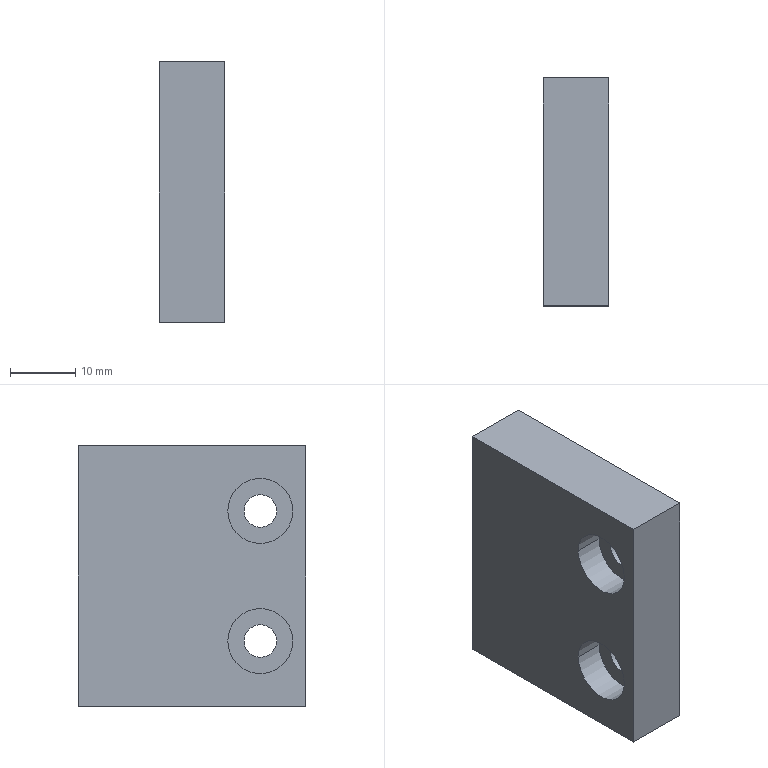Component | SolidWorks | SYM0545-81-107-2 | 1 solid | 16 faces | box 10 x 35 x 40 mm | volume 13077 mm3 | cylinder 8 | plane 8 | commonest cylinder face diameters 10 x4 5 x4 | material PP Copolymer
build123d program:
from build123d import *

# Parameters (mm, degrees)
SKETCH2_W       = 40
SKETCH2_H       = 35
EXTRUDE1_DEPTH  = 10
SKETCH3_R       = 2.5
EXTRUDE3_DEPTH  = 42.533
SKETCH4_R       = 5
EXTRUDE4_DEPTH  = 4.5
LPATTERN1_COUNT = 2
LPATTERN1_PITCH = 20


with BuildPart() as part:
    # Sketch2 → Extrude1 (new body)
    with BuildSketch(Plane(origin=(0, 0, 0), x_dir=(1, 0, 0), z_dir=(0, 1, 0))):
        with Locations((0, -17.5)):
            Rectangle(SKETCH2_W, SKETCH2_H)
    extrude(amount=EXTRUDE1_DEPTH)

    # Sketch3 → Extrude3 (cut, through all)
    with BuildSketch(Plane(origin=(0, 0, 0), x_dir=(1, 0, 0), z_dir=(0, 1, 0))):
        with Locations(Location((-10, -28, 0), (0, 0, 270))):
            Circle(SKETCH3_R)
    extrude3 = extrude(amount=EXTRUDE3_DEPTH, mode=Mode.SUBTRACT)

    # Sketch4 → Extrude4 (cut)
    with BuildSketch(Plane(origin=(0, 10, 0), x_dir=(1, 0, 0), z_dir=(0, 1, 0))):
        with Locations(Location((-10, -28, 0), (0, 0, 270))):
            Circle(SKETCH4_R)
    extrude4 = extrude(amount=-EXTRUDE4_DEPTH, mode=Mode.SUBTRACT)

    # LPattern1: Extrude3, Extrude4 ×2
    with Locations(*[(i * LPATTERN1_PITCH, 0, 0) for i in range(1, LPATTERN1_COUNT)]):
        add(extrude3, mode=Mode.SUBTRACT)
        add(extrude4, mode=Mode.SUBTRACT)


solid = part.part

# Placed as in the assembly
solid = solid.moved(Location((322.251, 468.143, 1010.518), (90, 0, 90)))
STEP:
#1=CARTESIAN_POINT('',(12.471,17.525,40.178));
#2=VERTEX_POINT('',#1);
#3=CARTESIAN_POINT('',(12.471,17.132,40.178));
#4=VERTEX_POINT('',#3);
#5=CARTESIAN_POINT('',(12.471,17.328,40.178));
#6=DIRECTION('',(-1.,0.,0.));
#7=DIRECTION('',(0.,-1.,0.));
#8=AXIS2_PLACEMENT_3D('',#5,#6,#7);
#9=CIRCLE('',#8,0.1969);
#10=EDGE_CURVE('',#2,#4,#9,.T.);
#11=ORIENTED_EDGE('',*,*,#10,.F.);
#12=CARTESIAN_POINT('',(12.293,17.525,40.178));
#13=VERTEX_POINT('',#12);
#14=CARTESIAN_POINT('',(12.471,17.525,40.178));
#15=DIRECTION('',(-1.,0.,0.));
#16=VECTOR('',#15,39.37);
#17=LINE('',#14,#16);
#18=EDGE_CURVE('',#2,#13,#17,.T.);
#19=ORIENTED_EDGE('',*,*,#18,.T.);
#20=CARTESIAN_POINT('',(12.293,17.132,40.178));
#21=VERTEX_POINT('',#20);
#22=CARTESIAN_POINT('',(12.293,17.328,40.178));
#23=DIRECTION('',(-1.,0.,0.));
#24=DIRECTION('',(0.,-1.,0.));
#25=AXIS2_PLACEMENT_3D('',#22,#23,#24);
#26=CIRCLE('',#25,0.1969);
#27=EDGE_CURVE('',#13,#21,#26,.T.);
#28=ORIENTED_EDGE('',*,*,#27,.T.);
#29=CARTESIAN_POINT('',(12.471,17.132,40.178));
#30=DIRECTION('',(-1.,0.,0.));
#31=VECTOR('',#30,39.37);
#32=LINE('',#29,#31);
#33=EDGE_CURVE('',#4,#21,#32,.T.);
#34=ORIENTED_EDGE('',*,*,#33,.F.);
#35=EDGE_LOOP('',(#11,#19,#28,#34));
#36=FACE_OUTER_BOUND('',#35,.T.);
#37=CARTESIAN_POINT('',(12.471,17.328,40.178));
#38=DIRECTION('',(-1.,0.,0.));
#39=DIRECTION('',(0.,-1.,0.));
#40=AXIS2_PLACEMENT_3D('',#37,#38,#39);
#41=CYLINDRICAL_SURFACE('',#40,0.1969);
#42=ADVANCED_FACE('',(#36),#41,.F.);
#43=CARTESIAN_POINT('',(12.471,17.525,39.39));
#44=VERTEX_POINT('',#43);
#45=CARTESIAN_POINT('',(12.471,17.132,39.39));
#46=VERTEX_POINT('',#45);
#47=CARTESIAN_POINT('',(12.471,17.328,39.39));
#48=DIRECTION('',(-1.,0.,0.));
#49=DIRECTION('',(0.,-1.,0.));
#50=AXIS2_PLACEMENT_3D('',#47,#48,#49);
#51=CIRCLE('',#50,0.1969);
#52=EDGE_CURVE('',#44,#46,#51,.T.);
#53=ORIENTED_EDGE('',*,*,#52,.F.);
#54=CARTESIAN_POINT('',(12.293,17.525,39.39));
#55=VERTEX_POINT('',#54);
#56=CARTESIAN_POINT('',(12.471,17.525,39.39));
#57=DIRECTION('',(-1.,0.,0.));
#58=VECTOR('',#57,39.37);
#59=LINE('',#56,#58);
#60=EDGE_CURVE('',#44,#55,#59,.T.);
#61=ORIENTED_EDGE('',*,*,#60,.T.);
#62=CARTESIAN_POINT('',(12.293,17.132,39.39));
#63=VERTEX_POINT('',#62);
#64=CARTESIAN_POINT('',(12.293,17.328,39.39));
#65=DIRECTION('',(-1.,0.,0.));
#66=DIRECTION('',(0.,-1.,0.));
#67=AXIS2_PLACEMENT_3D('',#64,#65,#66);
#68=CIRCLE('',#67,0.1969);
#69=EDGE_CURVE('',#55,#63,#68,.T.);
#70=ORIENTED_EDGE('',*,*,#69,.T.);
#71=CARTESIAN_POINT('',(12.471,17.132,39.39));
#72=DIRECTION('',(-1.,0.,0.));
#73=VECTOR('',#72,39.37);
#74=LINE('',#71,#73);
#75=EDGE_CURVE('',#46,#63,#74,.T.);
#76=ORIENTED_EDGE('',*,*,#75,.F.);
#77=EDGE_LOOP('',(#53,#61,#70,#76));
#78=FACE_OUTER_BOUND('',#77,.T.);
#79=CARTESIAN_POINT('',(12.471,17.328,39.39));
#80=DIRECTION('',(-1.,0.,0.));
#81=DIRECTION('',(0.,-1.,0.));
#82=AXIS2_PLACEMENT_3D('',#79,#80,#81);
#83=CYLINDRICAL_SURFACE('',#82,0.1969);
#84=ADVANCED_FACE('',(#78),#83,.F.);
#85=CARTESIAN_POINT('',(12.471,17.427,39.39));
#86=VERTEX_POINT('',#85);
#87=CARTESIAN_POINT('',(12.471,17.23,39.39));
#88=VERTEX_POINT('',#87);
#89=CARTESIAN_POINT('',(12.471,17.328,39.39));
#90=DIRECTION('',(-1.,0.,0.));
#91=DIRECTION('',(0.,-1.,0.));
#92=AXIS2_PLACEMENT_3D('',#89,#90,#91);
#93=CIRCLE('',#92,0.09843);
#94=EDGE_CURVE('',#86,#88,#93,.T.);
#95=ORIENTED_EDGE('',*,*,#94,.T.);
#96=CARTESIAN_POINT('',(12.687,17.23,39.39));
#97=VERTEX_POINT('',#96);
#98=CARTESIAN_POINT('',(12.293,17.23,39.39));
#99=DIRECTION('',(1.,-0.,-0.));
#100=VECTOR('',#99,39.37);
#101=LINE('',#98,#100);
#102=EDGE_CURVE('',#88,#97,#101,.T.);
#103=ORIENTED_EDGE('',*,*,#102,.T.);
#104=CARTESIAN_POINT('',(12.687,17.427,39.39));
#105=VERTEX_POINT('',#104);
#106=CARTESIAN_POINT('',(12.687,17.328,39.39));
#107=DIRECTION('',(-1.,0.,0.));
#108=DIRECTION('',(0.,-1.,0.));
#109=AXIS2_PLACEMENT_3D('',#106,#107,#108);
#110=CIRCLE('',#109,0.09843);
#111=EDGE_CURVE('',#105,#97,#110,.T.);
#112=ORIENTED_EDGE('',*,*,#111,.F.);
#113=CARTESIAN_POINT('',(12.293,17.427,39.39));
#114=DIRECTION('',(1.,-0.,-0.));
#115=VECTOR('',#114,39.37);
#116=LINE('',#113,#115);
#117=EDGE_CURVE('',#86,#105,#116,.T.);
#118=ORIENTED_EDGE('',*,*,#117,.F.);
#119=EDGE_LOOP('',(#95,#103,#112,#118));
#120=FACE_OUTER_BOUND('',#119,.T.);
#121=CARTESIAN_POINT('',(12.293,17.328,39.39));
#122=DIRECTION('',(1.,-0.,-0.));
#123=DIRECTION('',(0.,1.,0.));
#124=AXIS2_PLACEMENT_3D('',#121,#122,#123);
#125=CYLINDRICAL_SURFACE('',#124,0.09843);
#126=ADVANCED_FACE('',(#120),#125,.F.);
#127=CARTESIAN_POINT('',(12.471,17.427,40.178));
#128=VERTEX_POINT('',#127);
#129=CARTESIAN_POINT('',(12.471,17.23,40.178));
#130=VERTEX_POINT('',#129);
#131=CARTESIAN_POINT('',(12.471,17.328,40.178));
#132=DIRECTION('',(-1.,0.,0.));
#133=DIRECTION('',(0.,-1.,0.));
#134=AXIS2_PLACEMENT_3D('',#131,#132,#133);
#135=CIRCLE('',#134,0.09843);
#136=EDGE_CURVE('',#128,#130,#135,.T.);
#137=ORIENTED_EDGE('',*,*,#136,.T.);
#138=CARTESIAN_POINT('',(12.687,17.23,40.178));
#139=VERTEX_POINT('',#138);
#140=CARTESIAN_POINT('',(12.293,17.23,40.178));
#141=DIRECTION('',(1.,-0.,-0.));
#142=VECTOR('',#141,39.37);
#143=LINE('',#140,#142);
#144=EDGE_CURVE('',#130,#139,#143,.T.);
#145=ORIENTED_EDGE('',*,*,#144,.T.);
#146=CARTESIAN_POINT('',(12.687,17.427,40.178));
#147=VERTEX_POINT('',#146);
#148=CARTESIAN_POINT('',(12.687,17.328,40.178));
#149=DIRECTION('',(-1.,0.,0.));
#150=DIRECTION('',(0.,-1.,0.));
#151=AXIS2_PLACEMENT_3D('',#148,#149,#150);
#152=CIRCLE('',#151,0.09843);
#153=EDGE_CURVE('',#147,#139,#152,.T.);
#154=ORIENTED_EDGE('',*,*,#153,.F.);
#155=CARTESIAN_POINT('',(12.293,17.427,40.178));
#156=DIRECTION('',(1.,-0.,-0.));
#157=VECTOR('',#156,39.37);
#158=LINE('',#155,#157);
#159=EDGE_CURVE('',#128,#147,#158,.T.);
#160=ORIENTED_EDGE('',*,*,#159,.F.);
#161=EDGE_LOOP('',(#137,#145,#154,#160));
#162=FACE_OUTER_BOUND('',#161,.T.);
#163=CARTESIAN_POINT('',(12.293,17.328,40.178));
#164=DIRECTION('',(1.,-0.,-0.));
#165=DIRECTION('',(0.,1.,0.));
#166=AXIS2_PLACEMENT_3D('',#163,#164,#165);
#167=CYLINDRICAL_SURFACE('',#166,0.09843);
#168=ADVANCED_FACE('',(#162),#167,.F.);
#169=ORIENTED_EDGE('',*,*,#144,.F.);
#170=CARTESIAN_POINT('',(12.471,17.328,40.178));
#171=DIRECTION('',(-1.,0.,0.));
#172=DIRECTION('',(0.,-1.,0.));
#173=AXIS2_PLACEMENT_3D('',#170,#171,#172);
#174=CIRCLE('',#173,0.09843);
#175=EDGE_CURVE('',#130,#128,#174,.T.);
#176=ORIENTED_EDGE('',*,*,#175,.T.);
#177=ORIENTED_EDGE('',*,*,#159,.T.);
#178=CARTESIAN_POINT('',(12.687,17.328,40.178));
#179=DIRECTION('',(-1.,0.,0.));
#180=DIRECTION('',(0.,-1.,0.));
#181=AXIS2_PLACEMENT_3D('',#178,#179,#180);
#182=CIRCLE('',#181,0.09843);
#183=EDGE_CURVE('',#139,#147,#182,.T.);
#184=ORIENTED_EDGE('',*,*,#183,.F.);
#185=EDGE_LOOP('',(#169,#176,#177,#184));
#186=FACE_OUTER_BOUND('',#185,.T.);
#187=CARTESIAN_POINT('',(12.293,17.328,40.178));
#188=DIRECTION('',(1.,-0.,-0.));
#189=DIRECTION('',(0.,1.,0.));
#190=AXIS2_PLACEMENT_3D('',#187,#188,#189);
#191=CYLINDRICAL_SURFACE('',#190,0.09843);
#192=ADVANCED_FACE('',(#186),#191,.F.);
#193=CARTESIAN_POINT('',(12.293,17.328,40.178));
#194=DIRECTION('',(-1.,0.,0.));
#195=DIRECTION('',(0.,-1.,0.));
#196=AXIS2_PLACEMENT_3D('',#193,#194,#195);
#197=CIRCLE('',#196,0.1969);
#198=EDGE_CURVE('',#21,#13,#197,.T.);
#199=ORIENTED_EDGE('',*,*,#198,.F.);
#200=ORIENTED_EDGE('',*,*,#27,.F.);
#201=EDGE_LOOP('',(#199,#200));
#202=FACE_BOUND('',#201,.T.);
#203=CARTESIAN_POINT('',(12.293,18.431,38.997));
#204=VERTEX_POINT('',#203);
#205=CARTESIAN_POINT('',(12.293,17.053,38.997));
#206=VERTEX_POINT('',#205);
#207=CARTESIAN_POINT('',(12.293,18.431,38.997));
#208=DIRECTION('',(-0.,-1.,0.));
#209=VECTOR('',#208,39.37);
#210=LINE('',#207,#209);
#211=EDGE_CURVE('',#204,#206,#210,.T.);
#212=ORIENTED_EDGE('',*,*,#211,.T.);
#213=CARTESIAN_POINT('',(12.293,17.053,40.572));
#214=VERTEX_POINT('',#213);
#215=CARTESIAN_POINT('',(12.293,17.053,38.997));
#216=DIRECTION('',(0.,0.,1.));
#217=VECTOR('',#216,39.37);
#218=LINE('',#215,#217);
#219=EDGE_CURVE('',#206,#214,#218,.T.);
#220=ORIENTED_EDGE('',*,*,#219,.T.);
#221=CARTESIAN_POINT('',(12.293,18.431,40.572));
#222=VERTEX_POINT('',#221);
#223=CARTESIAN_POINT('',(12.293,18.431,40.572));
#224=DIRECTION('',(0.,1.,-0.));
#225=VECTOR('',#224,39.37);
#226=LINE('',#223,#225);
#227=EDGE_CURVE('',#214,#222,#226,.T.);
#228=ORIENTED_EDGE('',*,*,#227,.T.);
#229=CARTESIAN_POINT('',(12.293,18.431,38.997));
#230=DIRECTION('',(-0.,-0.,-1.));
#231=VECTOR('',#230,39.37);
#232=LINE('',#229,#231);
#233=EDGE_CURVE('',#222,#204,#232,.T.);
#234=ORIENTED_EDGE('',*,*,#233,.T.);
#235=EDGE_LOOP('',(#212,#220,#228,#234));
#236=FACE_OUTER_BOUND('',#235,.T.);
#237=CARTESIAN_POINT('',(12.293,17.328,39.39));
#238=DIRECTION('',(-1.,0.,0.));
#239=DIRECTION('',(0.,-1.,0.));
#240=AXIS2_PLACEMENT_3D('',#237,#238,#239);
#241=CIRCLE('',#240,0.1969);
#242=EDGE_CURVE('',#63,#55,#241,.T.);
#243=ORIENTED_EDGE('',*,*,#242,.F.);
#244=ORIENTED_EDGE('',*,*,#69,.F.);
#245=EDGE_LOOP('',(#243,#244));
#246=FACE_BOUND('',#245,.T.);
#247=CARTESIAN_POINT('',(12.293,17.053,38.997));
#248=DIRECTION('',(-1.,0.,0.));
#249=DIRECTION('',(-0.,-1.,0.));
#250=AXIS2_PLACEMENT_3D('',#247,#248,#249);
#251=PLANE('',#250);
#252=ADVANCED_FACE('',(#202,#236,#246),#251,.T.);
#253=ORIENTED_EDGE('',*,*,#111,.T.);
#254=CARTESIAN_POINT('',(12.687,17.328,39.39));
#255=DIRECTION('',(-1.,0.,0.));
#256=DIRECTION('',(0.,-1.,0.));
#257=AXIS2_PLACEMENT_3D('',#254,#255,#256);
#258=CIRCLE('',#257,0.09843);
#259=EDGE_CURVE('',#97,#105,#258,.T.);
#260=ORIENTED_EDGE('',*,*,#259,.T.);
#261=EDGE_LOOP('',(#253,#260));
#262=FACE_BOUND('',#261,.T.);
#263=CARTESIAN_POINT('',(12.687,18.431,38.997));
#264=VERTEX_POINT('',#263);
#265=CARTESIAN_POINT('',(12.687,17.053,38.997));
#266=VERTEX_POINT('',#265);
#267=CARTESIAN_POINT('',(12.687,18.431,38.997));
#268=DIRECTION('',(-0.,-1.,0.));
#269=VECTOR('',#268,39.37);
#270=LINE('',#267,#269);
#271=EDGE_CURVE('',#264,#266,#270,.T.);
#272=ORIENTED_EDGE('',*,*,#271,.F.);
#273=CARTESIAN_POINT('',(12.687,18.431,40.572));
#274=VERTEX_POINT('',#273);
#275=CARTESIAN_POINT('',(12.687,18.431,38.997));
#276=DIRECTION('',(-0.,-0.,-1.));
#277=VECTOR('',#276,39.37);
#278=LINE('',#275,#277);
#279=EDGE_CURVE('',#274,#264,#278,.T.);
#280=ORIENTED_EDGE('',*,*,#279,.F.);
#281=CARTESIAN_POINT('',(12.687,17.053,40.572));
#282=VERTEX_POINT('',#281);
#283=CARTESIAN_POINT('',(12.687,18.431,40.572));
#284=DIRECTION('',(0.,1.,-0.));
#285=VECTOR('',#284,39.37);
#286=LINE('',#283,#285);
#287=EDGE_CURVE('',#282,#274,#286,.T.);
#288=ORIENTED_EDGE('',*,*,#287,.F.);
#289=CARTESIAN_POINT('',(12.687,17.053,38.997));
#290=DIRECTION('',(0.,0.,1.));
#291=VECTOR('',#290,39.37);
#292=LINE('',#289,#291);
#293=EDGE_CURVE('',#266,#282,#292,.T.);
#294=ORIENTED_EDGE('',*,*,#293,.F.);
#295=EDGE_LOOP('',(#272,#280,#288,#294));
#296=FACE_OUTER_BOUND('',#295,.T.);
#297=ORIENTED_EDGE('',*,*,#153,.T.);
#298=ORIENTED_EDGE('',*,*,#183,.T.);
#299=EDGE_LOOP('',(#297,#298));
#300=FACE_BOUND('',#299,.T.);
#301=CARTESIAN_POINT('',(12.687,17.053,38.997));
#302=DIRECTION('',(-1.,0.,0.));
#303=DIRECTION('',(-0.,-1.,0.));
#304=AXIS2_PLACEMENT_3D('',#301,#302,#303);
#305=PLANE('',#304);
#306=ADVANCED_FACE('',(#262,#296,#300),#305,.F.);
#307=ORIENTED_EDGE('',*,*,#102,.F.);
#308=CARTESIAN_POINT('',(12.471,17.328,39.39));
#309=DIRECTION('',(-1.,0.,0.));
#310=DIRECTION('',(0.,-1.,0.));
#311=AXIS2_PLACEMENT_3D('',#308,#309,#310);
#312=CIRCLE('',#311,0.09843);
#313=EDGE_CURVE('',#88,#86,#312,.T.);
#314=ORIENTED_EDGE('',*,*,#313,.T.);
#315=ORIENTED_EDGE('',*,*,#117,.T.);
#316=ORIENTED_EDGE('',*,*,#259,.F.);
#317=EDGE_LOOP('',(#307,#314,#315,#316));
#318=FACE_OUTER_BOUND('',#317,.T.);
#319=CARTESIAN_POINT('',(12.293,17.328,39.39));
#320=DIRECTION('',(1.,-0.,-0.));
#321=DIRECTION('',(0.,1.,0.));
#322=AXIS2_PLACEMENT_3D('',#319,#320,#321);
#323=CYLINDRICAL_SURFACE('',#322,0.09843);
#324=ADVANCED_FACE('',(#318),#323,.F.);
#325=ORIENTED_EDGE('',*,*,#271,.T.);
#326=CARTESIAN_POINT('',(12.293,17.053,38.997));
#327=DIRECTION('',(1.,-0.,-0.));
#328=VECTOR('',#327,39.37);
#329=LINE('',#326,#328);
#330=EDGE_CURVE('',#206,#266,#329,.T.);
#331=ORIENTED_EDGE('',*,*,#330,.F.);
#332=ORIENTED_EDGE('',*,*,#211,.F.);
#333=CARTESIAN_POINT('',(12.293,18.431,38.997));
#334=DIRECTION('',(1.,-0.,-0.));
#335=VECTOR('',#334,39.37);
#336=LINE('',#333,#335);
#337=EDGE_CURVE('',#204,#264,#336,.T.);
#338=ORIENTED_EDGE('',*,*,#337,.T.);
#339=EDGE_LOOP('',(#325,#331,#332,#338));
#340=FACE_OUTER_BOUND('',#339,.T.);
#341=CARTESIAN_POINT('',(12.293,18.431,38.997));
#342=DIRECTION('',(0.,0.,1.));
#343=DIRECTION('',(0.,1.,-0.));
#344=AXIS2_PLACEMENT_3D('',#341,#342,#343);
#345=PLANE('',#344);
#346=ADVANCED_FACE('',(#340),#345,.F.);
#347=ORIENTED_EDGE('',*,*,#293,.T.);
#348=CARTESIAN_POINT('',(12.293,17.053,40.572));
#349=DIRECTION('',(1.,-0.,-0.));
#350=VECTOR('',#349,39.37);
#351=LINE('',#348,#350);
#352=EDGE_CURVE('',#214,#282,#351,.T.);
#353=ORIENTED_EDGE('',*,*,#352,.F.);
#354=ORIENTED_EDGE('',*,*,#219,.F.);
#355=ORIENTED_EDGE('',*,*,#330,.T.);
#356=EDGE_LOOP('',(#347,#353,#354,#355));
#357=FACE_OUTER_BOUND('',#356,.T.);
#358=CARTESIAN_POINT('',(12.293,17.053,38.997));
#359=DIRECTION('',(0.,1.,-0.));
#360=DIRECTION('',(-0.,-0.,-1.));
#361=AXIS2_PLACEMENT_3D('',#358,#359,#360);
#362=PLANE('',#361);
#363=ADVANCED_FACE('',(#357),#362,.F.);
#364=ORIENTED_EDGE('',*,*,#287,.T.);
#365=CARTESIAN_POINT('',(12.293,18.431,40.572));
#366=DIRECTION('',(1.,-0.,-0.));
#367=VECTOR('',#366,39.37);
#368=LINE('',#365,#367);
#369=EDGE_CURVE('',#222,#274,#368,.T.);
#370=ORIENTED_EDGE('',*,*,#369,.F.);
#371=ORIENTED_EDGE('',*,*,#227,.F.);
#372=ORIENTED_EDGE('',*,*,#352,.T.);
#373=EDGE_LOOP('',(#364,#370,#371,#372));
#374=FACE_OUTER_BOUND('',#373,.T.);
#375=CARTESIAN_POINT('',(12.293,18.431,40.572));
#376=DIRECTION('',(-0.,-0.,-1.));
#377=DIRECTION('',(-0.,-1.,0.));
#378=AXIS2_PLACEMENT_3D('',#375,#376,#377);
#379=PLANE('',#378);
#380=ADVANCED_FACE('',(#374),#379,.F.);
#381=ORIENTED_EDGE('',*,*,#279,.T.);
#382=ORIENTED_EDGE('',*,*,#337,.F.);
#383=ORIENTED_EDGE('',*,*,#233,.F.);
#384=ORIENTED_EDGE('',*,*,#369,.T.);
#385=EDGE_LOOP('',(#381,#382,#383,#384));
#386=FACE_OUTER_BOUND('',#385,.T.);
#387=CARTESIAN_POINT('',(12.293,18.431,38.997));
#388=DIRECTION('',(-0.,-1.,0.));
#389=DIRECTION('',(0.,0.,1.));
#390=AXIS2_PLACEMENT_3D('',#387,#388,#389);
#391=PLANE('',#390);
#392=ADVANCED_FACE('',(#386),#391,.F.);
#393=ORIENTED_EDGE('',*,*,#60,.F.);
#394=CARTESIAN_POINT('',(12.471,17.328,39.39));
#395=DIRECTION('',(-1.,0.,0.));
#396=DIRECTION('',(0.,-1.,0.));
#397=AXIS2_PLACEMENT_3D('',#394,#395,#396);
#398=CIRCLE('',#397,0.1969);
#399=EDGE_CURVE('',#46,#44,#398,.T.);
#400=ORIENTED_EDGE('',*,*,#399,.F.);
#401=ORIENTED_EDGE('',*,*,#75,.T.);
#402=ORIENTED_EDGE('',*,*,#242,.T.);
#403=EDGE_LOOP('',(#393,#400,#401,#402));
#404=FACE_OUTER_BOUND('',#403,.T.);
#405=CARTESIAN_POINT('',(12.471,17.328,39.39));
#406=DIRECTION('',(-1.,0.,0.));
#407=DIRECTION('',(0.,-1.,0.));
#408=AXIS2_PLACEMENT_3D('',#405,#406,#407);
#409=CYLINDRICAL_SURFACE('',#408,0.1969);
#410=ADVANCED_FACE('',(#404),#409,.F.);
#411=ORIENTED_EDGE('',*,*,#94,.F.);
#412=ORIENTED_EDGE('',*,*,#313,.F.);
#413=EDGE_LOOP('',(#411,#412));
#414=FACE_BOUND('',#413,.T.);
#415=ORIENTED_EDGE('',*,*,#399,.T.);
#416=ORIENTED_EDGE('',*,*,#52,.T.);
#417=EDGE_LOOP('',(#415,#416));
#418=FACE_OUTER_BOUND('',#417,.T.);
#419=CARTESIAN_POINT('',(12.471,17.328,39.39));
#420=DIRECTION('',(-1.,0.,0.));
#421=DIRECTION('',(-0.,-1.,0.));
#422=AXIS2_PLACEMENT_3D('',#419,#420,#421);
#423=PLANE('',#422);
#424=ADVANCED_FACE('',(#414,#418),#423,.T.);
#425=ORIENTED_EDGE('',*,*,#18,.F.);
#426=CARTESIAN_POINT('',(12.471,17.328,40.178));
#427=DIRECTION('',(-1.,0.,0.));
#428=DIRECTION('',(0.,-1.,0.));
#429=AXIS2_PLACEMENT_3D('',#426,#427,#428);
#430=CIRCLE('',#429,0.1969);
#431=EDGE_CURVE('',#4,#2,#430,.T.);
#432=ORIENTED_EDGE('',*,*,#431,.F.);
#433=ORIENTED_EDGE('',*,*,#33,.T.);
#434=ORIENTED_EDGE('',*,*,#198,.T.);
#435=EDGE_LOOP('',(#425,#432,#433,#434));
#436=FACE_OUTER_BOUND('',#435,.T.);
#437=CARTESIAN_POINT('',(12.471,17.328,40.178));
#438=DIRECTION('',(-1.,0.,0.));
#439=DIRECTION('',(0.,-1.,0.));
#440=AXIS2_PLACEMENT_3D('',#437,#438,#439);
#441=CYLINDRICAL_SURFACE('',#440,0.1969);
#442=ADVANCED_FACE('',(#436),#441,.F.);
#443=ORIENTED_EDGE('',*,*,#136,.F.);
#444=ORIENTED_EDGE('',*,*,#175,.F.);
#445=EDGE_LOOP('',(#443,#444));
#446=FACE_BOUND('',#445,.T.);
#447=ORIENTED_EDGE('',*,*,#431,.T.);
#448=ORIENTED_EDGE('',*,*,#10,.T.);
#449=EDGE_LOOP('',(#447,#448));
#450=FACE_OUTER_BOUND('',#449,.T.);
#451=CARTESIAN_POINT('',(12.471,17.328,40.178));
#452=DIRECTION('',(-1.,0.,0.));
#453=DIRECTION('',(-0.,-1.,0.));
#454=AXIS2_PLACEMENT_3D('',#451,#452,#453);
#455=PLANE('',#454);
#456=ADVANCED_FACE('',(#446,#450),#455,.T.);
#457=CLOSED_SHELL('',(#42,#84,#126,#168,#192,#252,#306,#324,#346,#363,#380,#392,#410,#424,#442,#456));
#458=MANIFOLD_SOLID_BREP('',#457);
#459=CARTESIAN_POINT('',(0.,0.,0.));
#460=DIRECTION('',(0.,0.,1.));
#461=DIRECTION('',(1.,0.,0.));
#462=AXIS2_PLACEMENT_3D('',#459,#460,#461);
#463=(LENGTH_UNIT()NAMED_UNIT(*)SI_UNIT($,.METRE.));
#464=LENGTH_MEASURE_WITH_UNIT(LENGTH_MEASURE(0.0254),#463);
#465=DIMENSIONAL_EXPONENTS(1.,0.,0.,0.,0.,0.,0.);
#466=(CONVERSION_BASED_UNIT('',#464)LENGTH_UNIT()NAMED_UNIT(#465));
#467=UNCERTAINTY_MEASURE_WITH_UNIT(LENGTH_MEASURE(0.00001),#466,'','');
#468=(NAMED_UNIT(*)PLANE_ANGLE_UNIT()SI_UNIT($,.RADIAN.));
#469=(NAMED_UNIT(*)SI_UNIT($,.STERADIAN.)SOLID_ANGLE_UNIT());
#470=(GEOMETRIC_REPRESENTATION_CONTEXT(3)GLOBAL_UNCERTAINTY_ASSIGNED_CONTEXT((#467))GLOBAL_UNIT_ASSIGNED_CONTEXT((#466,#468,#469))REPRESENTATION_CONTEXT('',''));
#471=ADVANCED_BREP_SHAPE_REPRESENTATION('',(#458,#462),#470);
#472=COLOUR_RGB('',0.7922,0.8196,0.9333);
#473=FILL_AREA_STYLE_COLOUR('',#472);
#474=FILL_AREA_STYLE('',(#473));
#475=SURFACE_STYLE_FILL_AREA(#474);
#476=SURFACE_SIDE_STYLE('',(#475));
#477=SURFACE_STYLE_USAGE(.BOTH.,#476);
#478=PRESENTATION_STYLE_ASSIGNMENT((#477));
#479=STYLED_ITEM('',(#478),#458);
#480=PRESENTATION_LAYER_ASSIGNMENT('','',(#479));
#481=(LENGTH_UNIT()NAMED_UNIT(*)SI_UNIT($,.METRE.));
#482=LENGTH_MEASURE_WITH_UNIT(LENGTH_MEASURE(0.0254),#481);
#483=DIMENSIONAL_EXPONENTS(1.,0.,0.,0.,0.,0.,0.);
#484=(CONVERSION_BASED_UNIT('',#482)LENGTH_UNIT()NAMED_UNIT(#483));
#485=UNCERTAINTY_MEASURE_WITH_UNIT(LENGTH_MEASURE(0.00001),#484,'','');
#486=(NAMED_UNIT(*)PLANE_ANGLE_UNIT()SI_UNIT($,.RADIAN.));
#487=(NAMED_UNIT(*)SI_UNIT($,.STERADIAN.)SOLID_ANGLE_UNIT());
#488=(GEOMETRIC_REPRESENTATION_CONTEXT(3)GLOBAL_UNCERTAINTY_ASSIGNED_CONTEXT((#485))GLOBAL_UNIT_ASSIGNED_CONTEXT((#484,#486,#487))REPRESENTATION_CONTEXT('',''));
#489=MECHANICAL_DESIGN_GEOMETRIC_PRESENTATION_REPRESENTATION('',(#479),#488);